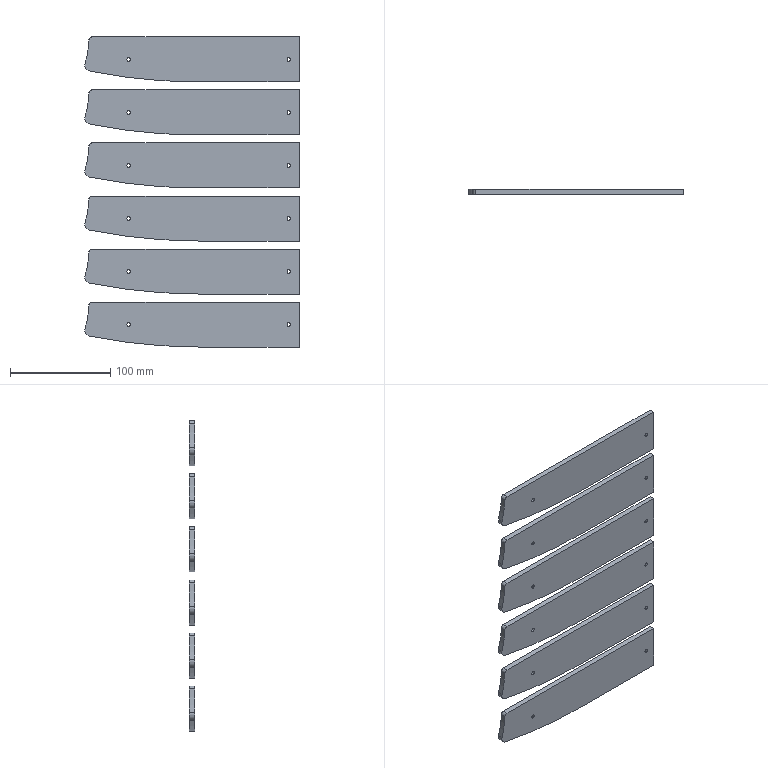CAM job | Mastercam | mm | 4 operations | part box 214.46 x 5 x 310
1. Contour (Ramp) | 3 - 3 平铣刀
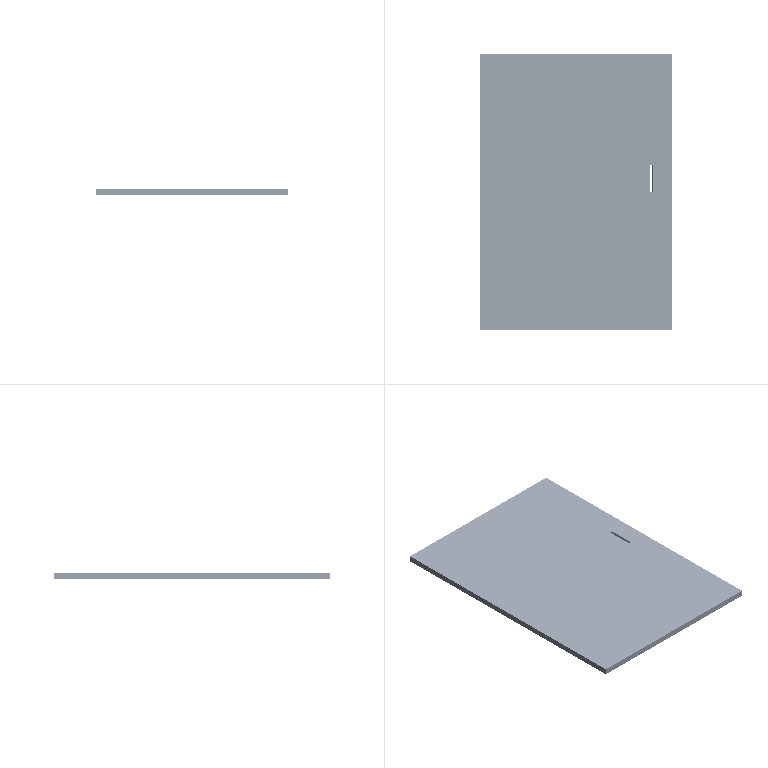2. Contour (2D chamfer) | 7 - 4 倒角刀
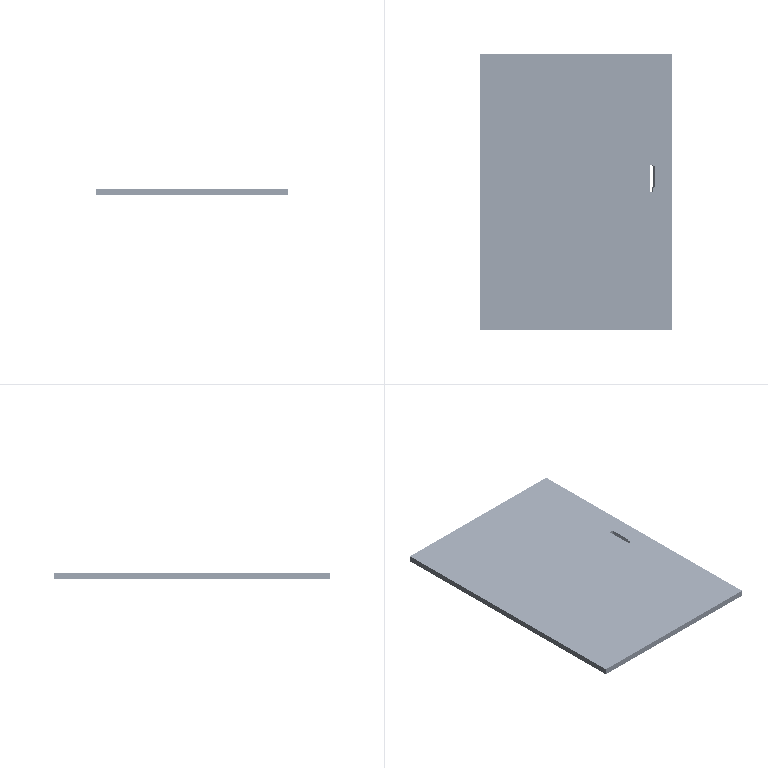3. Drill/Counterbore | 7 - 4 倒角刀
4. Contour (Ramp) | 2 - 2 平铣刀